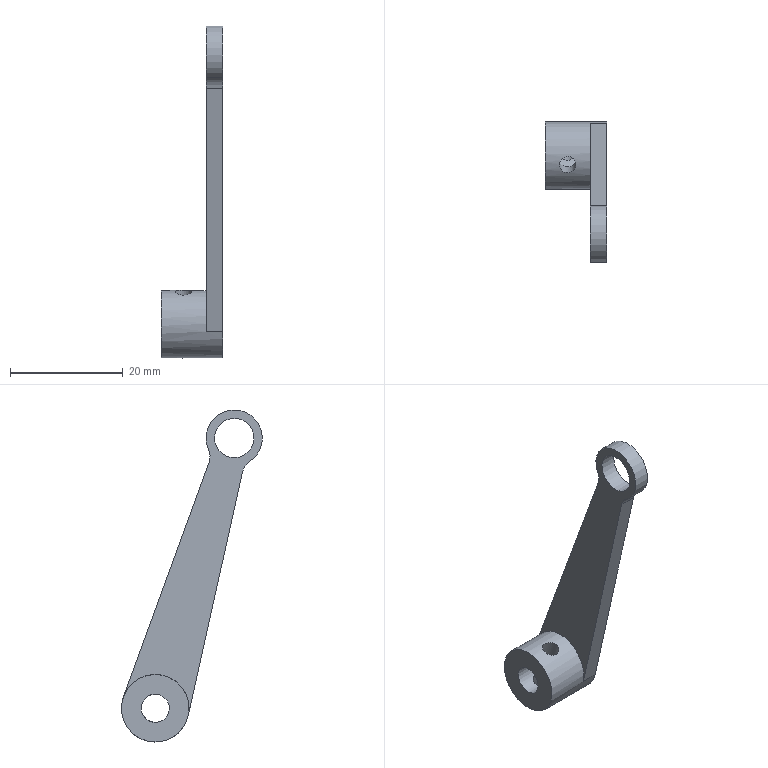Component | NX | 23C__27 | 1 solid | 13 faces | volume 2161 mm3 | cylinder 8 | plane 5 | commonest cylinder face diameters 6 x2 3 x2 12 x1 5 x1 10 x1 7 x1